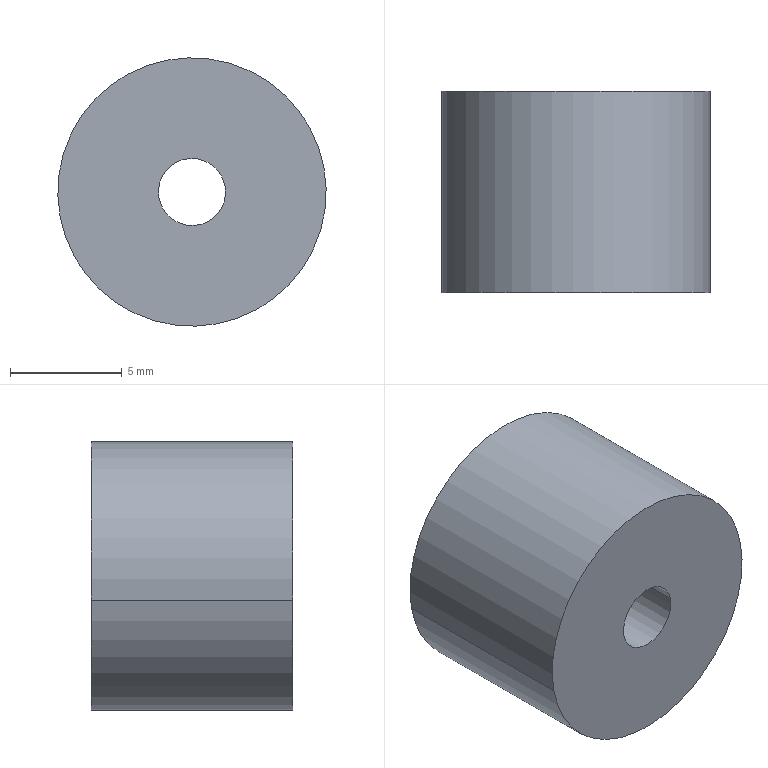Component | SolidWorks | RubberBufferPad-1 | 1 solid | 9 faces | box 12 x 9 x 12 mm | volume 879 mm3 | cylinder 6 | plane 3 | commonest cylinder face diameters 5 x2 12 x2 3 x2
build123d program:
from build123d import *

# Parameters (mm, degrees)
SKETCH2_R           = 6
SKETCH2_R_2         = 1.5
BOSS_EXTRUDE1_DEPTH = 9
SKETCH3_R           = 2.5
CUT_EXTRUDE1_DEPTH  = 6


with BuildPart() as part:
    # Sketch2 → Boss-Extrude1 (new body)
    with BuildSketch(Plane.XY):
        with Locations((64, -354)):
            Circle(SKETCH2_R)
        with Locations((64, -354)):
            Circle(SKETCH2_R_2, mode=Mode.SUBTRACT)
    extrude(amount=BOSS_EXTRUDE1_DEPTH)

    # Sketch3 → Cut-Extrude1 (cut)
    with BuildSketch(Plane.XY.offset(9)):
        with Locations((64, -354)):
            Circle(SKETCH3_R)
    extrude(amount=-CUT_EXTRUDE1_DEPTH, mode=Mode.SUBTRACT)


solid = part.part

# Placed as in the assembly
solid = solid.moved(Location((-563.947, -147.651, 0), (-90, 0, 0)))
STEP:
#1=CARTESIAN_POINT('',(-19.586,-5.695,13.955));
#2=VERTEX_POINT('',#1);
#3=CARTESIAN_POINT('',(-19.78,-5.695,13.919));
#4=VERTEX_POINT('',#3);
#5=CARTESIAN_POINT('',(-19.683,-5.695,13.937));
#6=DIRECTION('',(0.,1.,0.));
#7=DIRECTION('',(-0.9837,0.,-0.18));
#8=AXIS2_PLACEMENT_3D('',#5,#6,#7);
#9=CIRCLE('',#8,0.09843);
#10=EDGE_CURVE('',#2,#4,#9,.T.);
#11=ORIENTED_EDGE('',*,*,#10,.F.);
#12=CARTESIAN_POINT('',(-19.586,-5.459,13.955));
#13=VERTEX_POINT('',#12);
#14=CARTESIAN_POINT('',(-19.586,-5.695,13.955));
#15=DIRECTION('',(0.,1.,0.));
#16=VECTOR('',#15,39.37);
#17=LINE('',#14,#16);
#18=EDGE_CURVE('',#2,#13,#17,.T.);
#19=ORIENTED_EDGE('',*,*,#18,.T.);
#20=CARTESIAN_POINT('',(-19.78,-5.459,13.919));
#21=VERTEX_POINT('',#20);
#22=CARTESIAN_POINT('',(-19.683,-5.459,13.937));
#23=DIRECTION('',(0.,1.,0.));
#24=DIRECTION('',(-0.9837,0.,-0.18));
#25=AXIS2_PLACEMENT_3D('',#22,#23,#24);
#26=CIRCLE('',#25,0.09843);
#27=EDGE_CURVE('',#13,#21,#26,.T.);
#28=ORIENTED_EDGE('',*,*,#27,.T.);
#29=CARTESIAN_POINT('',(-19.78,-5.695,13.919));
#30=DIRECTION('',(0.,1.,0.));
#31=VECTOR('',#30,39.37);
#32=LINE('',#29,#31);
#33=EDGE_CURVE('',#4,#21,#32,.T.);
#34=ORIENTED_EDGE('',*,*,#33,.F.);
#35=EDGE_LOOP('',(#11,#19,#28,#34));
#36=FACE_OUTER_BOUND('',#35,.T.);
#37=CARTESIAN_POINT('',(-19.683,-5.695,13.937));
#38=DIRECTION('',(0.,1.,0.));
#39=DIRECTION('',(-0.9837,0.,-0.18));
#40=AXIS2_PLACEMENT_3D('',#37,#38,#39);
#41=CYLINDRICAL_SURFACE('',#40,0.09843);
#42=ADVANCED_FACE('',(#36),#41,.F.);
#43=CARTESIAN_POINT('',(-19.915,-5.459,13.894));
#44=VERTEX_POINT('',#43);
#45=CARTESIAN_POINT('',(-19.451,-5.459,13.98));
#46=VERTEX_POINT('',#45);
#47=CARTESIAN_POINT('',(-19.683,-5.459,13.937));
#48=DIRECTION('',(0.,1.,0.));
#49=DIRECTION('',(-0.9837,0.,-0.18));
#50=AXIS2_PLACEMENT_3D('',#47,#48,#49);
#51=CIRCLE('',#50,0.2362);
#52=EDGE_CURVE('',#44,#46,#51,.T.);
#53=ORIENTED_EDGE('',*,*,#52,.F.);
#54=CARTESIAN_POINT('',(-19.915,-5.813,13.894));
#55=VERTEX_POINT('',#54);
#56=CARTESIAN_POINT('',(-19.915,-5.459,13.894));
#57=DIRECTION('',(-0.,-1.,-0.));
#58=VECTOR('',#57,39.37);
#59=LINE('',#56,#58);
#60=EDGE_CURVE('',#44,#55,#59,.T.);
#61=ORIENTED_EDGE('',*,*,#60,.T.);
#62=CARTESIAN_POINT('',(-19.451,-5.813,13.98));
#63=VERTEX_POINT('',#62);
#64=CARTESIAN_POINT('',(-19.683,-5.813,13.937));
#65=DIRECTION('',(0.,1.,0.));
#66=DIRECTION('',(-0.9837,0.,-0.18));
#67=AXIS2_PLACEMENT_3D('',#64,#65,#66);
#68=CIRCLE('',#67,0.2362);
#69=EDGE_CURVE('',#55,#63,#68,.T.);
#70=ORIENTED_EDGE('',*,*,#69,.T.);
#71=CARTESIAN_POINT('',(-19.451,-5.459,13.98));
#72=DIRECTION('',(-0.,-1.,-0.));
#73=VECTOR('',#72,39.37);
#74=LINE('',#71,#73);
#75=EDGE_CURVE('',#46,#63,#74,.T.);
#76=ORIENTED_EDGE('',*,*,#75,.F.);
#77=EDGE_LOOP('',(#53,#61,#70,#76));
#78=FACE_OUTER_BOUND('',#77,.T.);
#79=CARTESIAN_POINT('',(-19.683,-5.459,13.937));
#80=DIRECTION('',(-0.,-1.,-0.));
#81=DIRECTION('',(0.9837,0.,0.18));
#82=AXIS2_PLACEMENT_3D('',#79,#80,#81);
#83=CYLINDRICAL_SURFACE('',#82,0.2362);
#84=ADVANCED_FACE('',(#78),#83,.T.);
#85=CARTESIAN_POINT('',(-19.625,-5.695,13.948));
#86=VERTEX_POINT('',#85);
#87=CARTESIAN_POINT('',(-19.741,-5.695,13.926));
#88=VERTEX_POINT('',#87);
#89=CARTESIAN_POINT('',(-19.683,-5.695,13.937));
#90=DIRECTION('',(0.,1.,0.));
#91=DIRECTION('',(-0.9837,0.,-0.18));
#92=AXIS2_PLACEMENT_3D('',#89,#90,#91);
#93=CIRCLE('',#92,0.05906);
#94=EDGE_CURVE('',#86,#88,#93,.T.);
#95=ORIENTED_EDGE('',*,*,#94,.T.);
#96=CARTESIAN_POINT('',(-19.741,-5.813,13.926));
#97=VERTEX_POINT('',#96);
#98=CARTESIAN_POINT('',(-19.741,-5.459,13.926));
#99=DIRECTION('',(-0.,-1.,-0.));
#100=VECTOR('',#99,39.37);
#101=LINE('',#98,#100);
#102=EDGE_CURVE('',#88,#97,#101,.T.);
#103=ORIENTED_EDGE('',*,*,#102,.T.);
#104=CARTESIAN_POINT('',(-19.625,-5.813,13.948));
#105=VERTEX_POINT('',#104);
#106=CARTESIAN_POINT('',(-19.683,-5.813,13.937));
#107=DIRECTION('',(0.,1.,0.));
#108=DIRECTION('',(-0.9837,0.,-0.18));
#109=AXIS2_PLACEMENT_3D('',#106,#107,#108);
#110=CIRCLE('',#109,0.05906);
#111=EDGE_CURVE('',#105,#97,#110,.T.);
#112=ORIENTED_EDGE('',*,*,#111,.F.);
#113=CARTESIAN_POINT('',(-19.625,-5.459,13.948));
#114=DIRECTION('',(-0.,-1.,-0.));
#115=VECTOR('',#114,39.37);
#116=LINE('',#113,#115);
#117=EDGE_CURVE('',#86,#105,#116,.T.);
#118=ORIENTED_EDGE('',*,*,#117,.F.);
#119=EDGE_LOOP('',(#95,#103,#112,#118));
#120=FACE_OUTER_BOUND('',#119,.T.);
#121=CARTESIAN_POINT('',(-19.683,-5.459,13.937));
#122=DIRECTION('',(-0.,-1.,-0.));
#123=DIRECTION('',(0.9837,0.,0.18));
#124=AXIS2_PLACEMENT_3D('',#121,#122,#123);
#125=CYLINDRICAL_SURFACE('',#124,0.05906);
#126=ADVANCED_FACE('',(#120),#125,.F.);
#127=ORIENTED_EDGE('',*,*,#102,.F.);
#128=CARTESIAN_POINT('',(-19.683,-5.695,13.937));
#129=DIRECTION('',(0.,1.,0.));
#130=DIRECTION('',(-0.9837,0.,-0.18));
#131=AXIS2_PLACEMENT_3D('',#128,#129,#130);
#132=CIRCLE('',#131,0.05906);
#133=EDGE_CURVE('',#88,#86,#132,.T.);
#134=ORIENTED_EDGE('',*,*,#133,.T.);
#135=ORIENTED_EDGE('',*,*,#117,.T.);
#136=CARTESIAN_POINT('',(-19.683,-5.813,13.937));
#137=DIRECTION('',(0.,1.,0.));
#138=DIRECTION('',(-0.9837,0.,-0.18));
#139=AXIS2_PLACEMENT_3D('',#136,#137,#138);
#140=CIRCLE('',#139,0.05906);
#141=EDGE_CURVE('',#97,#105,#140,.T.);
#142=ORIENTED_EDGE('',*,*,#141,.F.);
#143=EDGE_LOOP('',(#127,#134,#135,#142));
#144=FACE_OUTER_BOUND('',#143,.T.);
#145=CARTESIAN_POINT('',(-19.683,-5.459,13.937));
#146=DIRECTION('',(-0.,-1.,-0.));
#147=DIRECTION('',(0.9837,0.,0.18));
#148=AXIS2_PLACEMENT_3D('',#145,#146,#147);
#149=CYLINDRICAL_SURFACE('',#148,0.05906);
#150=ADVANCED_FACE('',(#144),#149,.F.);
#151=CARTESIAN_POINT('',(-19.683,-5.459,13.937));
#152=DIRECTION('',(0.,1.,0.));
#153=DIRECTION('',(-0.9837,0.,-0.18));
#154=AXIS2_PLACEMENT_3D('',#151,#152,#153);
#155=CIRCLE('',#154,0.09843);
#156=EDGE_CURVE('',#21,#13,#155,.T.);
#157=ORIENTED_EDGE('',*,*,#156,.F.);
#158=ORIENTED_EDGE('',*,*,#27,.F.);
#159=EDGE_LOOP('',(#157,#158));
#160=FACE_BOUND('',#159,.T.);
#161=CARTESIAN_POINT('',(-19.683,-5.459,13.937));
#162=DIRECTION('',(0.,1.,0.));
#163=DIRECTION('',(-0.9837,0.,-0.18));
#164=AXIS2_PLACEMENT_3D('',#161,#162,#163);
#165=CIRCLE('',#164,0.2362);
#166=EDGE_CURVE('',#46,#44,#165,.T.);
#167=ORIENTED_EDGE('',*,*,#166,.T.);
#168=ORIENTED_EDGE('',*,*,#52,.T.);
#169=EDGE_LOOP('',(#167,#168));
#170=FACE_OUTER_BOUND('',#169,.T.);
#171=CARTESIAN_POINT('',(-19.683,-5.459,13.937));
#172=DIRECTION('',(0.,1.,0.));
#173=DIRECTION('',(-0.9837,0.,-0.18));
#174=AXIS2_PLACEMENT_3D('',#171,#172,#173);
#175=PLANE('',#174);
#176=ADVANCED_FACE('',(#160,#170),#175,.T.);
#177=CARTESIAN_POINT('',(-19.683,-5.813,13.937));
#178=DIRECTION('',(0.,1.,0.));
#179=DIRECTION('',(-0.9837,0.,-0.18));
#180=AXIS2_PLACEMENT_3D('',#177,#178,#179);
#181=CIRCLE('',#180,0.2362);
#182=EDGE_CURVE('',#63,#55,#181,.T.);
#183=ORIENTED_EDGE('',*,*,#182,.F.);
#184=ORIENTED_EDGE('',*,*,#69,.F.);
#185=EDGE_LOOP('',(#183,#184));
#186=FACE_OUTER_BOUND('',#185,.T.);
#187=ORIENTED_EDGE('',*,*,#111,.T.);
#188=ORIENTED_EDGE('',*,*,#141,.T.);
#189=EDGE_LOOP('',(#187,#188));
#190=FACE_BOUND('',#189,.T.);
#191=CARTESIAN_POINT('',(-19.683,-5.813,13.937));
#192=DIRECTION('',(0.,1.,0.));
#193=DIRECTION('',(-0.9837,0.,-0.18));
#194=AXIS2_PLACEMENT_3D('',#191,#192,#193);
#195=PLANE('',#194);
#196=ADVANCED_FACE('',(#186,#190),#195,.F.);
#197=ORIENTED_EDGE('',*,*,#60,.F.);
#198=ORIENTED_EDGE('',*,*,#166,.F.);
#199=ORIENTED_EDGE('',*,*,#75,.T.);
#200=ORIENTED_EDGE('',*,*,#182,.T.);
#201=EDGE_LOOP('',(#197,#198,#199,#200));
#202=FACE_OUTER_BOUND('',#201,.T.);
#203=CARTESIAN_POINT('',(-19.683,-5.459,13.937));
#204=DIRECTION('',(-0.,-1.,-0.));
#205=DIRECTION('',(0.9837,0.,0.18));
#206=AXIS2_PLACEMENT_3D('',#203,#204,#205);
#207=CYLINDRICAL_SURFACE('',#206,0.2362);
#208=ADVANCED_FACE('',(#202),#207,.T.);
#209=ORIENTED_EDGE('',*,*,#18,.F.);
#210=CARTESIAN_POINT('',(-19.683,-5.695,13.937));
#211=DIRECTION('',(0.,1.,0.));
#212=DIRECTION('',(-0.9837,0.,-0.18));
#213=AXIS2_PLACEMENT_3D('',#210,#211,#212);
#214=CIRCLE('',#213,0.09843);
#215=EDGE_CURVE('',#4,#2,#214,.T.);
#216=ORIENTED_EDGE('',*,*,#215,.F.);
#217=ORIENTED_EDGE('',*,*,#33,.T.);
#218=ORIENTED_EDGE('',*,*,#156,.T.);
#219=EDGE_LOOP('',(#209,#216,#217,#218));
#220=FACE_OUTER_BOUND('',#219,.T.);
#221=CARTESIAN_POINT('',(-19.683,-5.695,13.937));
#222=DIRECTION('',(0.,1.,0.));
#223=DIRECTION('',(-0.9837,0.,-0.18));
#224=AXIS2_PLACEMENT_3D('',#221,#222,#223);
#225=CYLINDRICAL_SURFACE('',#224,0.09843);
#226=ADVANCED_FACE('',(#220),#225,.F.);
#227=ORIENTED_EDGE('',*,*,#94,.F.);
#228=ORIENTED_EDGE('',*,*,#133,.F.);
#229=EDGE_LOOP('',(#227,#228));
#230=FACE_BOUND('',#229,.T.);
#231=ORIENTED_EDGE('',*,*,#215,.T.);
#232=ORIENTED_EDGE('',*,*,#10,.T.);
#233=EDGE_LOOP('',(#231,#232));
#234=FACE_OUTER_BOUND('',#233,.T.);
#235=CARTESIAN_POINT('',(-19.683,-5.695,13.937));
#236=DIRECTION('',(0.,1.,0.));
#237=DIRECTION('',(-0.9837,0.,-0.18));
#238=AXIS2_PLACEMENT_3D('',#235,#236,#237);
#239=PLANE('',#238);
#240=ADVANCED_FACE('',(#230,#234),#239,.T.);
#241=CLOSED_SHELL('',(#42,#84,#126,#150,#176,#196,#208,#226,#240));
#242=MANIFOLD_SOLID_BREP('',#241);
#243=CARTESIAN_POINT('',(0.,0.,0.));
#244=DIRECTION('',(0.,0.,1.));
#245=DIRECTION('',(1.,0.,0.));
#246=AXIS2_PLACEMENT_3D('',#243,#244,#245);
#247=(LENGTH_UNIT()NAMED_UNIT(*)SI_UNIT($,.METRE.));
#248=LENGTH_MEASURE_WITH_UNIT(LENGTH_MEASURE(0.0254),#247);
#249=DIMENSIONAL_EXPONENTS(1.,0.,0.,0.,0.,0.,0.);
#250=(CONVERSION_BASED_UNIT('',#248)LENGTH_UNIT()NAMED_UNIT(#249));
#251=UNCERTAINTY_MEASURE_WITH_UNIT(LENGTH_MEASURE(0.00001),#250,'','');
#252=(NAMED_UNIT(*)PLANE_ANGLE_UNIT()SI_UNIT($,.RADIAN.));
#253=(NAMED_UNIT(*)SI_UNIT($,.STERADIAN.)SOLID_ANGLE_UNIT());
#254=(GEOMETRIC_REPRESENTATION_CONTEXT(3)GLOBAL_UNCERTAINTY_ASSIGNED_CONTEXT((#251))GLOBAL_UNIT_ASSIGNED_CONTEXT((#250,#252,#253))REPRESENTATION_CONTEXT('',''));
#255=ADVANCED_BREP_SHAPE_REPRESENTATION('',(#242,#246),#254);
#256=COLOUR_RGB('',0.7922,0.8196,0.9333);
#257=FILL_AREA_STYLE_COLOUR('',#256);
#258=FILL_AREA_STYLE('',(#257));
#259=SURFACE_STYLE_FILL_AREA(#258);
#260=SURFACE_SIDE_STYLE('',(#259));
#261=SURFACE_STYLE_USAGE(.BOTH.,#260);
#262=PRESENTATION_STYLE_ASSIGNMENT((#261));
#263=STYLED_ITEM('',(#262),#242);
#264=PRESENTATION_LAYER_ASSIGNMENT('','',(#263));
#265=(LENGTH_UNIT()NAMED_UNIT(*)SI_UNIT($,.METRE.));
#266=LENGTH_MEASURE_WITH_UNIT(LENGTH_MEASURE(0.0254),#265);
#267=DIMENSIONAL_EXPONENTS(1.,0.,0.,0.,0.,0.,0.);
#268=(CONVERSION_BASED_UNIT('',#266)LENGTH_UNIT()NAMED_UNIT(#267));
#269=UNCERTAINTY_MEASURE_WITH_UNIT(LENGTH_MEASURE(0.00001),#268,'','');
#270=(NAMED_UNIT(*)PLANE_ANGLE_UNIT()SI_UNIT($,.RADIAN.));
#271=(NAMED_UNIT(*)SI_UNIT($,.STERADIAN.)SOLID_ANGLE_UNIT());
#272=(GEOMETRIC_REPRESENTATION_CONTEXT(3)GLOBAL_UNCERTAINTY_ASSIGNED_CONTEXT((#269))GLOBAL_UNIT_ASSIGNED_CONTEXT((#268,#270,#271))REPRESENTATION_CONTEXT('',''));
#273=MECHANICAL_DESIGN_GEOMETRIC_PRESENTATION_REPRESENTATION('',(#263),#272);